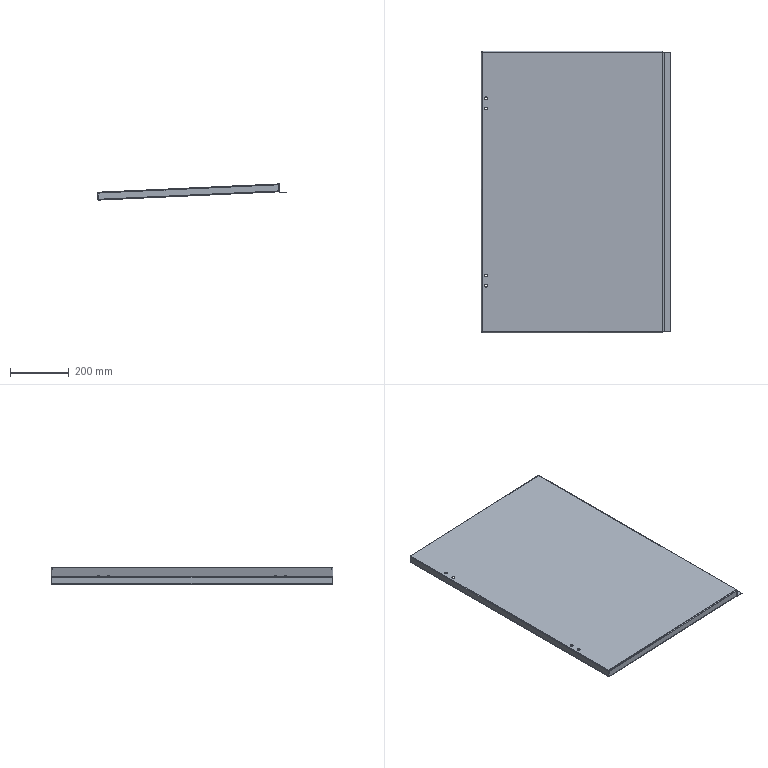Component | SolidWorks | 34LeftFront-2 | 1 solid | 78 faces | volume 1429387 mm3 | plane 46 | cylinder 24 | spline 8 | commonest cylinder face diameters 10 x8 2 x8 6 x8